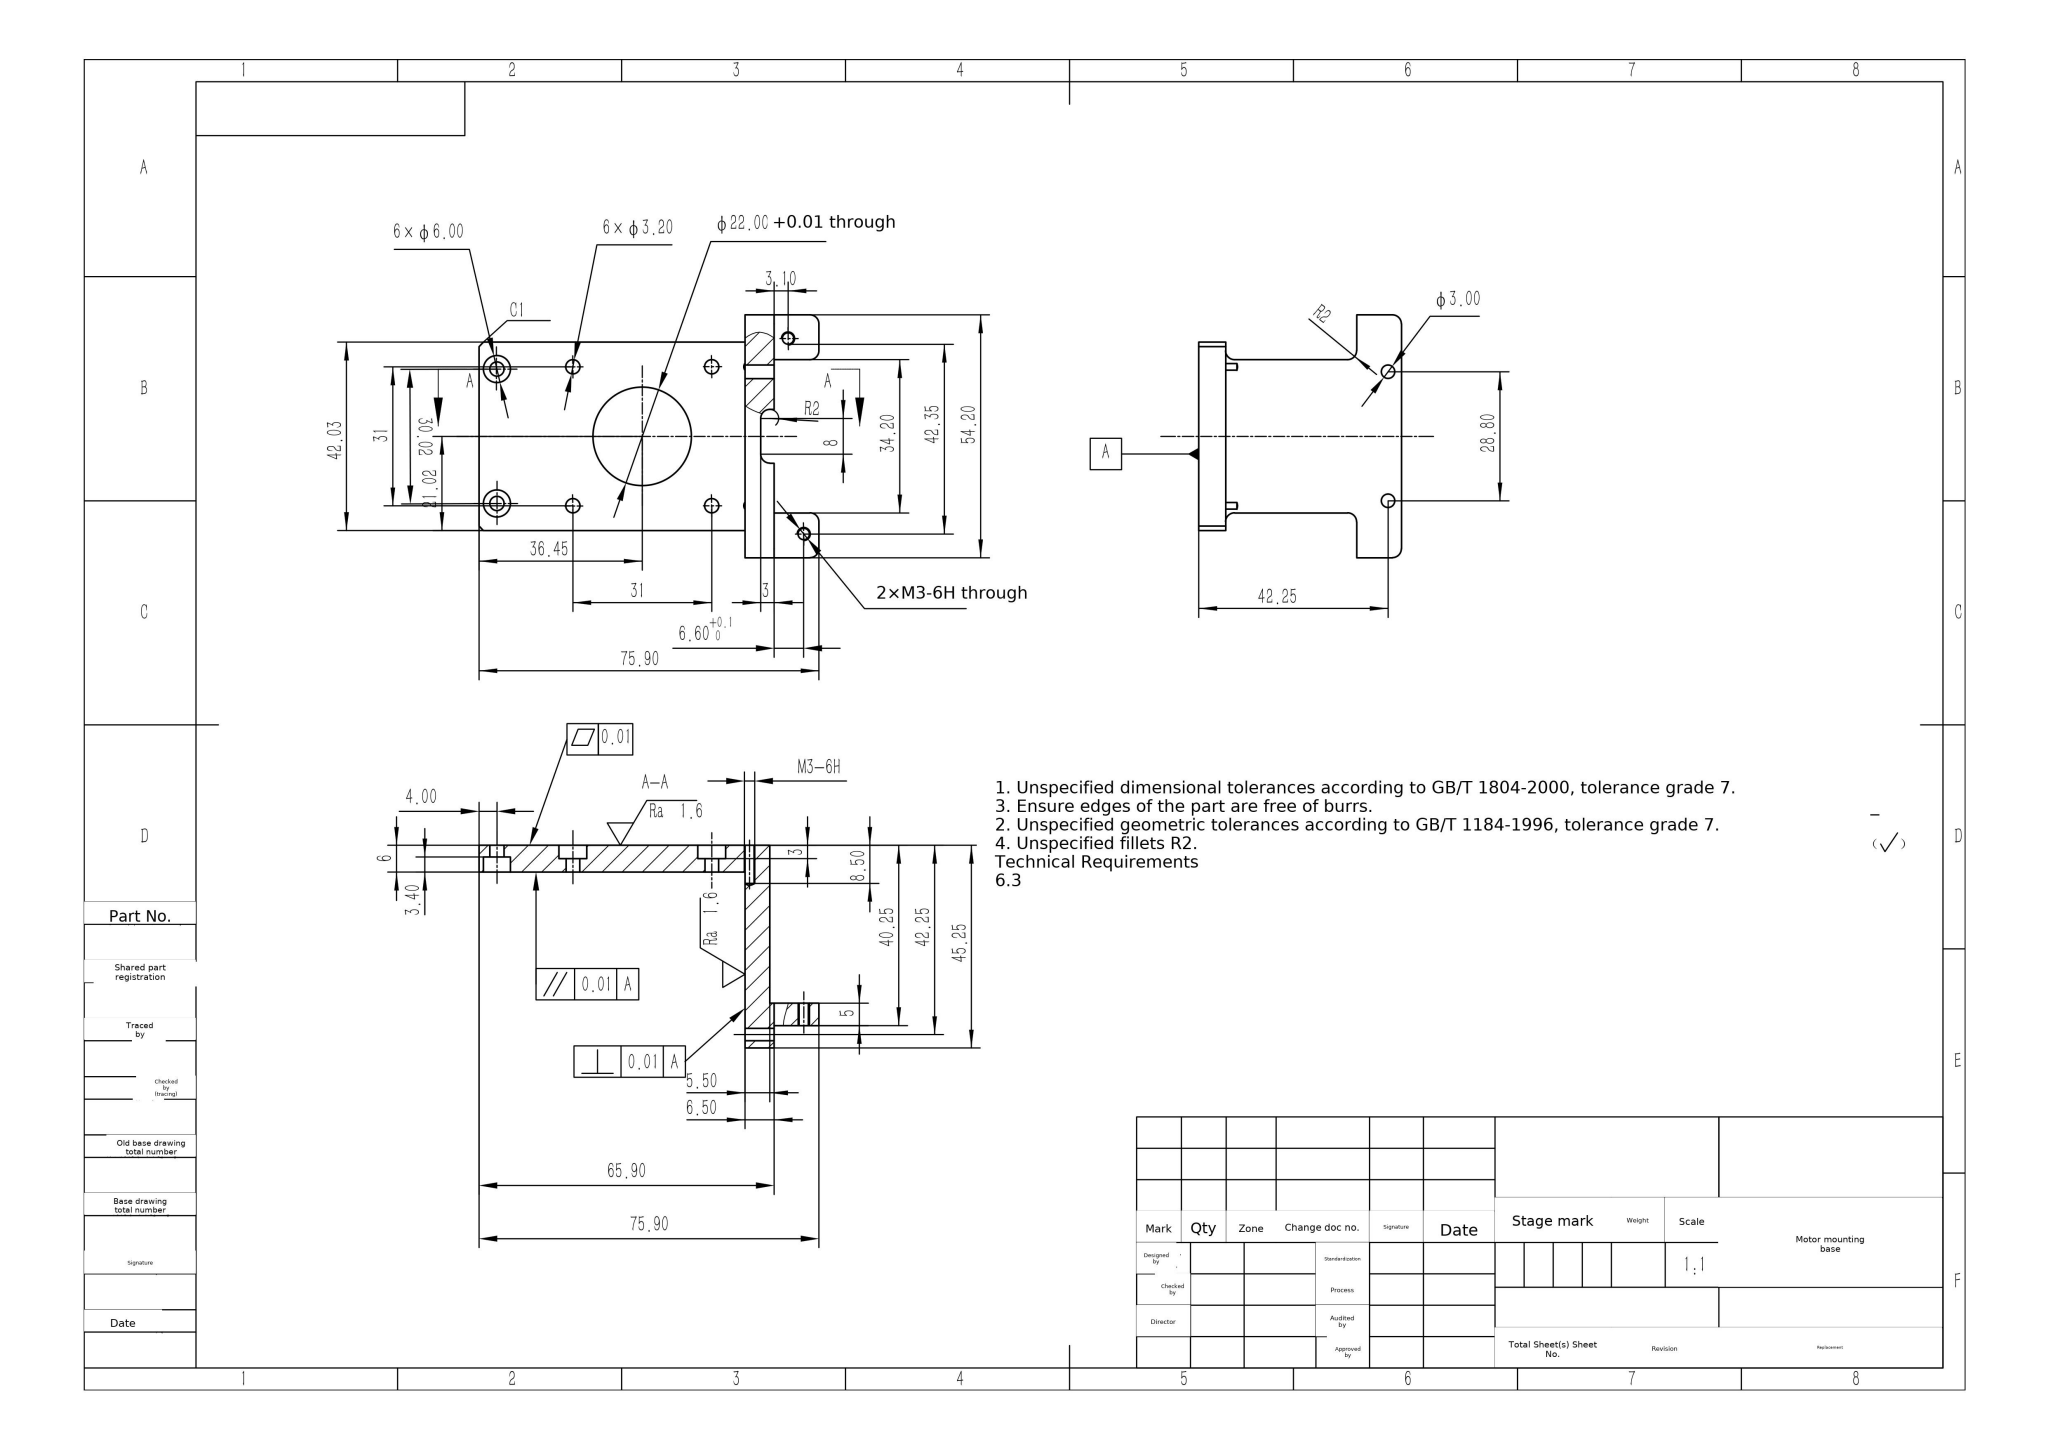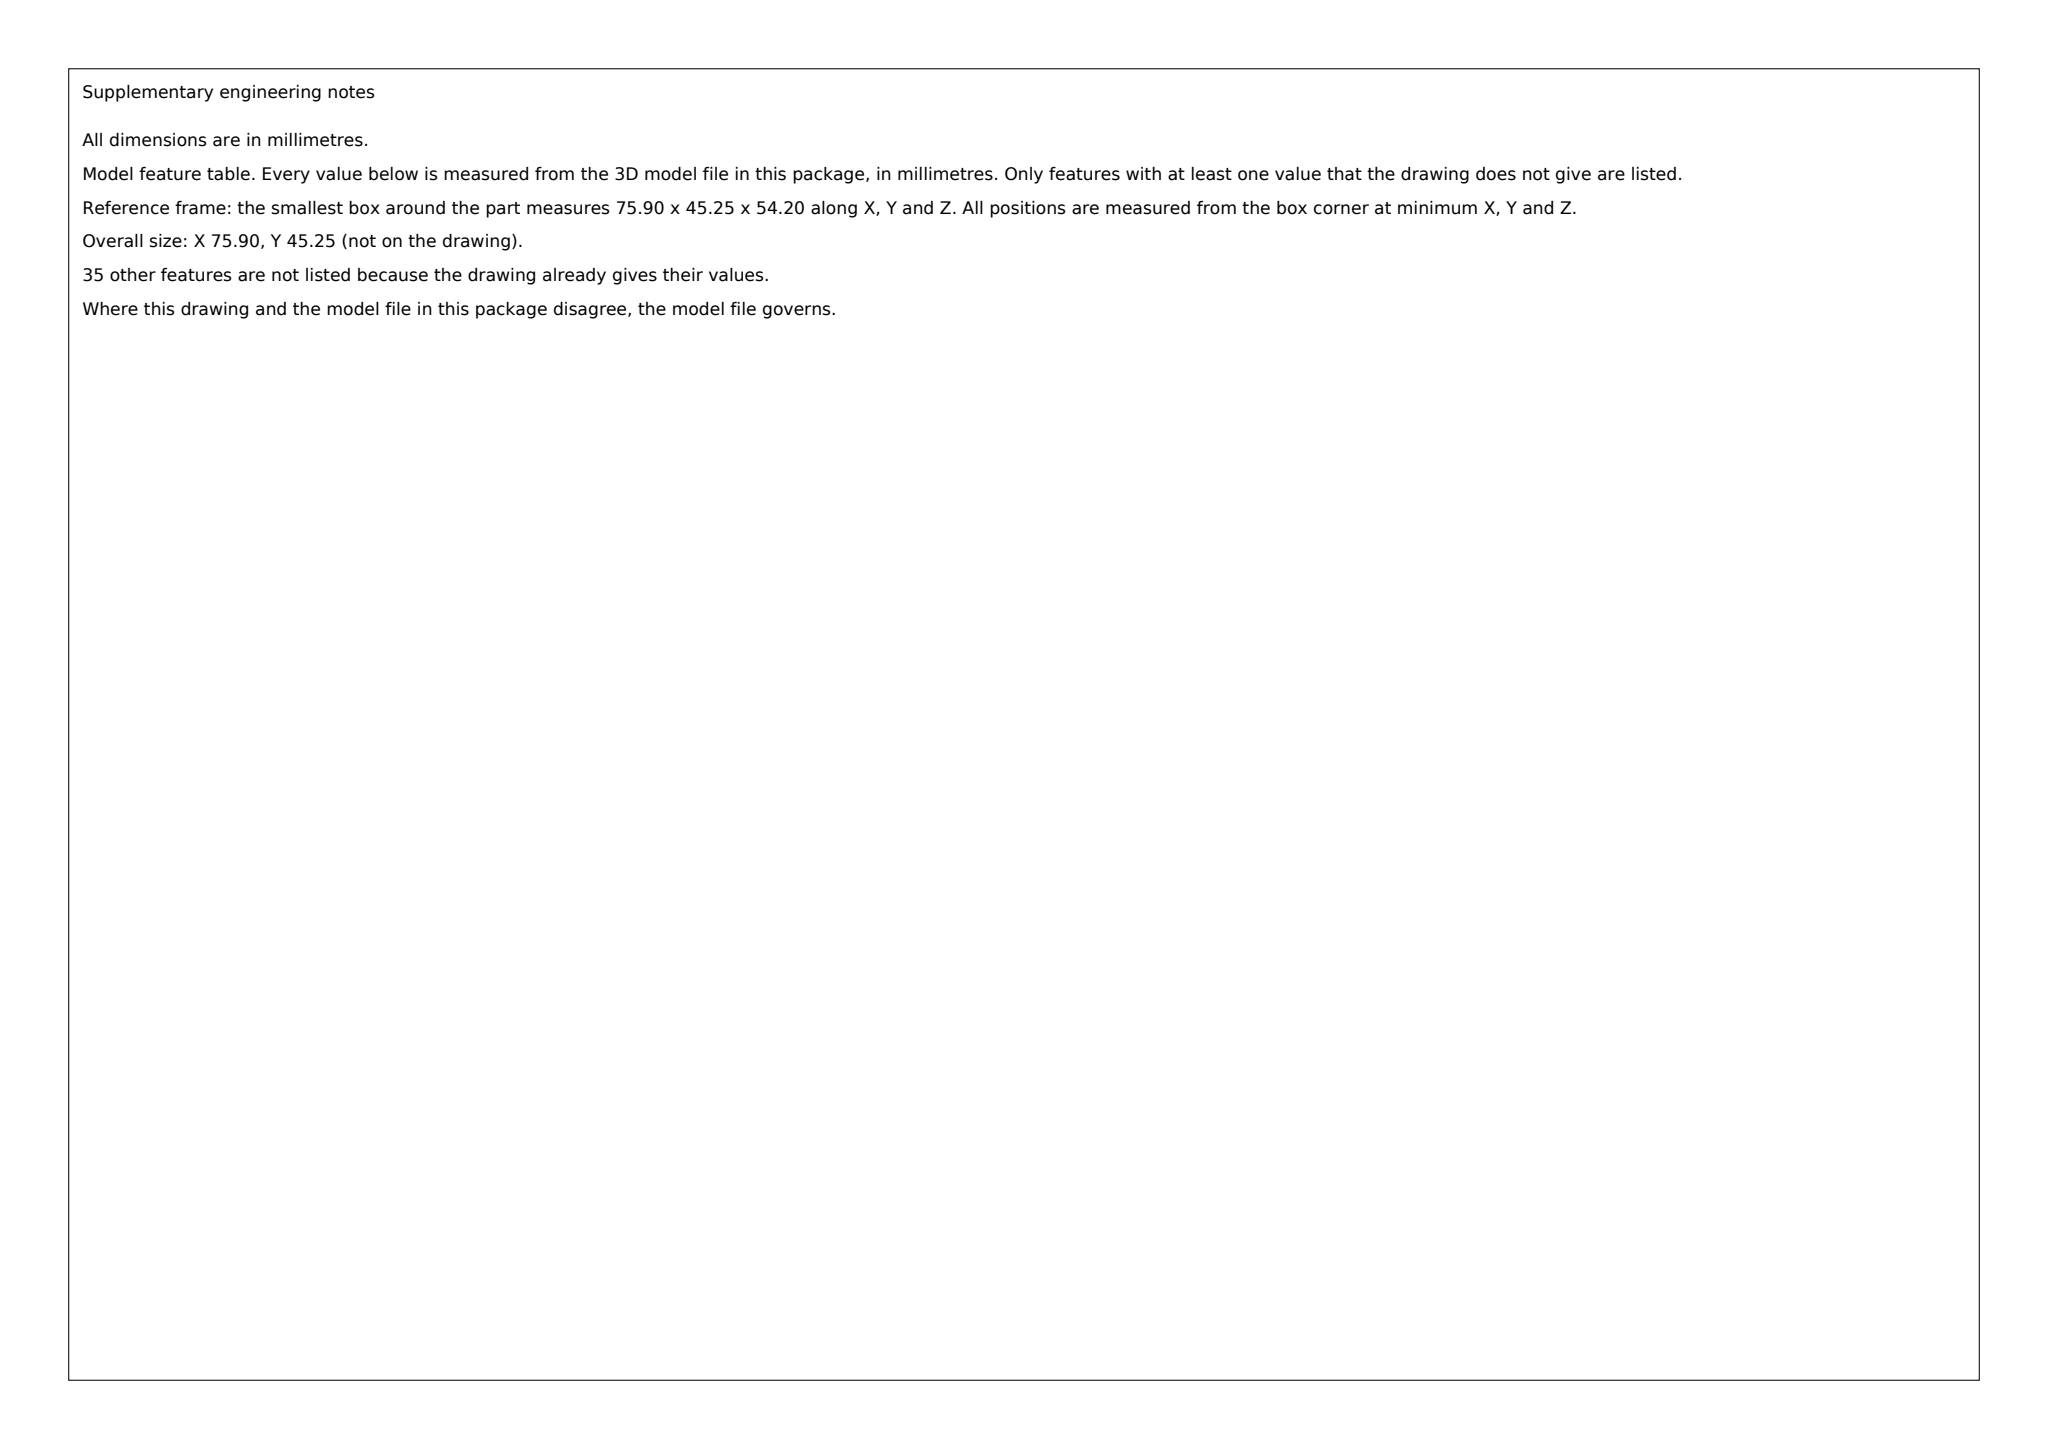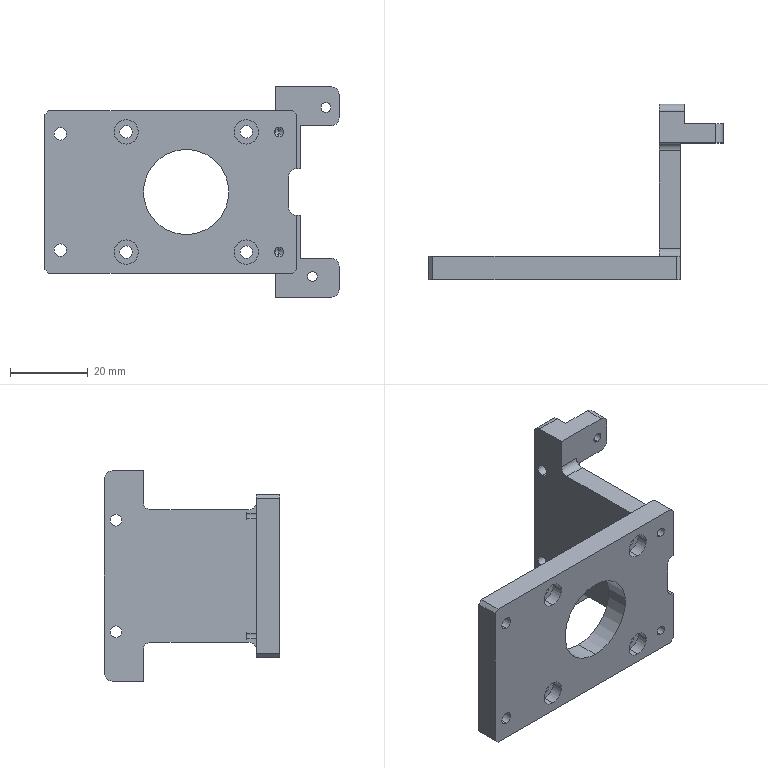Part | SolidWorks | mm | 1 solid | 90 faces | box 75.9 x 45.25 x 54.2 mm | volume 22031 mm3 | cylinder 50 | plane 36 | cone 4 | commonest cylinder face diameters 4 x12 3.2 x12 2.5 x8 6.3 x8 6 x4 3 x4 22 x2